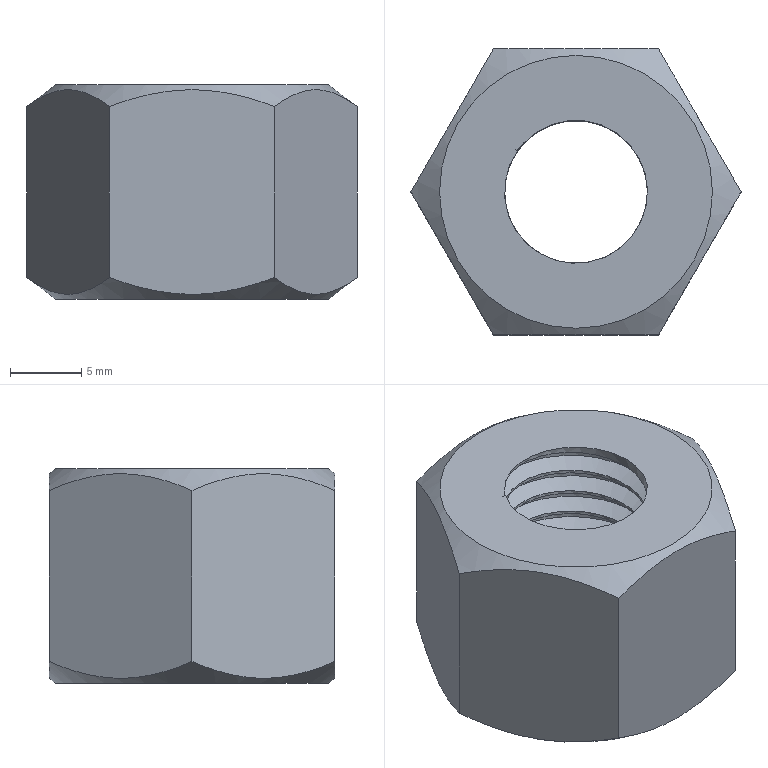Component | NX | 11__NUT_M10X1__2 | 1 solid | 15 faces | volume 3692 mm3 | plane 9 | cylinder 2 | cone 2 | spline 2 | commonest cylinder face diameters 10 x1 12 x1